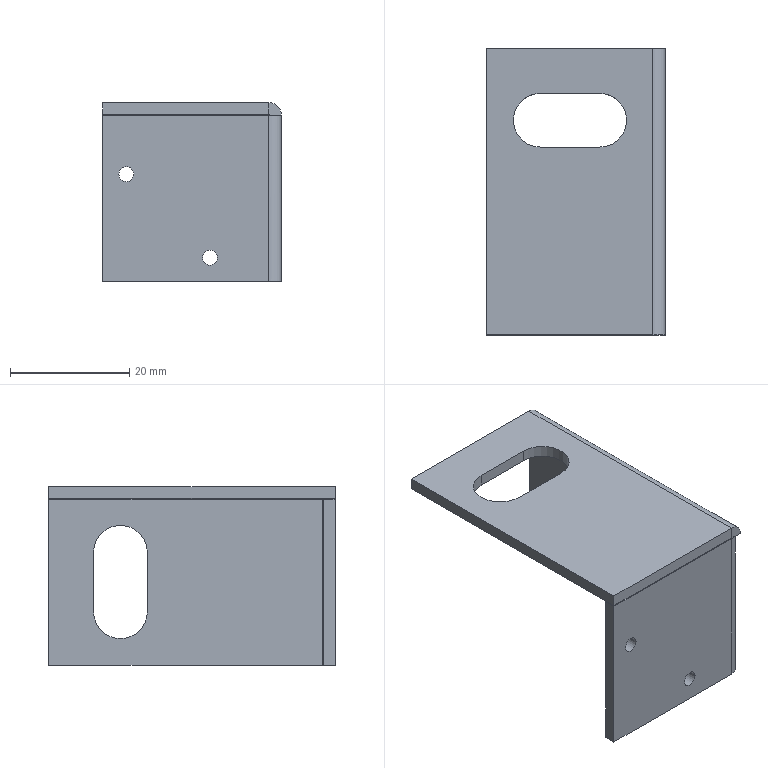Component | SolidWorks | LowerSealingPlateWeldingDrawingPG50-07-1_PG50-07-102(LowerCoverPlateWeldment2)-1 | 1 solid | 36 faces | box 30 x 48 x 30 mm | volume 6419 mm3 | plane 23 | cylinder 13 | commonest cylinder face diameters 9 x5 2.5 x4 0.3 x2 4.3 x2 | material AISI 1045 Steel, cold drawn
STEP:
#1=COLOUR_RGB('',0.7922,0.8196,0.9333);
#2=FILL_AREA_STYLE_COLOUR('',#1);
#3=FILL_AREA_STYLE('',(#2));
#4=SURFACE_STYLE_FILL_AREA(#3);
#5=SURFACE_SIDE_STYLE('',(#4));
#6=SURFACE_STYLE_USAGE(.BOTH.,#5);
#7=PRESENTATION_STYLE_ASSIGNMENT((#6));
#8=CARTESIAN_POINT('',(37.64,-11.134,13.484));
#9=VERTEX_POINT('',#8);
#10=CARTESIAN_POINT('',(37.542,-11.134,13.484));
#11=VERTEX_POINT('',#10);
#12=CARTESIAN_POINT('',(37.591,-11.134,13.484));
#13=DIRECTION('',(-0.,1.,0.));
#14=DIRECTION('',(-1.,0.,0.));
#15=AXIS2_PLACEMENT_3D('',#12,#13,#14);
#16=CIRCLE('',#15,0.04921);
#17=EDGE_CURVE('',#9,#11,#16,.T.);
#18=ORIENTED_EDGE('',*,*,#17,.F.);
#19=CARTESIAN_POINT('',(37.64,-11.055,13.484));
#20=VERTEX_POINT('',#19);
#21=CARTESIAN_POINT('',(37.64,-11.449,13.484));
#22=DIRECTION('',(0.,1.,0.));
#23=VECTOR('',#22,39.37);
#24=LINE('',#21,#23);
#25=EDGE_CURVE('',#9,#20,#24,.T.);
#26=ORIENTED_EDGE('',*,*,#25,.T.);
#27=CARTESIAN_POINT('',(37.542,-11.055,13.484));
#28=VERTEX_POINT('',#27);
#29=CARTESIAN_POINT('',(37.591,-11.055,13.484));
#30=DIRECTION('',(0.,1.,0.));
#31=DIRECTION('',(-1.,0.,0.));
#32=AXIS2_PLACEMENT_3D('',#29,#30,#31);
#33=CIRCLE('',#32,0.04921);
#34=EDGE_CURVE('',#20,#28,#33,.T.);
#35=ORIENTED_EDGE('',*,*,#34,.T.);
#36=CARTESIAN_POINT('',(37.542,-11.449,13.484));
#37=DIRECTION('',(0.,1.,0.));
#38=VECTOR('',#37,39.37);
#39=LINE('',#36,#38);
#40=EDGE_CURVE('',#11,#28,#39,.T.);
#41=ORIENTED_EDGE('',*,*,#40,.F.);
#42=EDGE_LOOP('',(#18,#26,#35,#41));
#43=FACE_OUTER_BOUND('',#42,.T.);
#44=CARTESIAN_POINT('',(37.591,-11.449,13.484));
#45=DIRECTION('',(0.,1.,0.));
#46=DIRECTION('',(-1.,0.,0.));
#47=AXIS2_PLACEMENT_3D('',#44,#45,#46);
#48=CYLINDRICAL_SURFACE('',#47,0.04921);
#49=ADVANCED_FACE('',(#43),#48,.F.);
#50=CARTESIAN_POINT('',(38.192,-11.134,12.933));
#51=VERTEX_POINT('',#50);
#52=CARTESIAN_POINT('',(38.093,-11.134,12.933));
#53=VERTEX_POINT('',#52);
#54=CARTESIAN_POINT('',(38.142,-11.134,12.933));
#55=DIRECTION('',(-0.,1.,0.));
#56=DIRECTION('',(-1.,0.,0.));
#57=AXIS2_PLACEMENT_3D('',#54,#55,#56);
#58=CIRCLE('',#57,0.04921);
#59=EDGE_CURVE('',#51,#53,#58,.T.);
#60=ORIENTED_EDGE('',*,*,#59,.F.);
#61=CARTESIAN_POINT('',(38.192,-11.055,12.933));
#62=VERTEX_POINT('',#61);
#63=CARTESIAN_POINT('',(38.192,-11.449,12.933));
#64=DIRECTION('',(0.,1.,0.));
#65=VECTOR('',#64,39.37);
#66=LINE('',#63,#65);
#67=EDGE_CURVE('',#51,#62,#66,.T.);
#68=ORIENTED_EDGE('',*,*,#67,.T.);
#69=CARTESIAN_POINT('',(38.093,-11.055,12.933));
#70=VERTEX_POINT('',#69);
#71=CARTESIAN_POINT('',(38.142,-11.055,12.933));
#72=DIRECTION('',(0.,1.,0.));
#73=DIRECTION('',(-1.,0.,0.));
#74=AXIS2_PLACEMENT_3D('',#71,#72,#73);
#75=CIRCLE('',#74,0.04921);
#76=EDGE_CURVE('',#62,#70,#75,.T.);
#77=ORIENTED_EDGE('',*,*,#76,.T.);
#78=CARTESIAN_POINT('',(38.093,-11.449,12.933));
#79=DIRECTION('',(0.,1.,0.));
#80=VECTOR('',#79,39.37);
#81=LINE('',#78,#80);
#82=EDGE_CURVE('',#53,#70,#81,.T.);
#83=ORIENTED_EDGE('',*,*,#82,.F.);
#84=EDGE_LOOP('',(#60,#68,#77,#83));
#85=FACE_OUTER_BOUND('',#84,.T.);
#86=CARTESIAN_POINT('',(38.142,-11.449,12.933));
#87=DIRECTION('',(0.,1.,0.));
#88=DIRECTION('',(-1.,0.,0.));
#89=AXIS2_PLACEMENT_3D('',#86,#87,#88);
#90=CYLINDRICAL_SURFACE('',#89,0.04921);
#91=ADVANCED_FACE('',(#85),#90,.F.);
#92=CARTESIAN_POINT('',(38.536,-9.539,13.13));
#93=VERTEX_POINT('',#92);
#94=CARTESIAN_POINT('',(38.536,-9.716,12.953));
#95=VERTEX_POINT('',#94);
#96=CARTESIAN_POINT('',(38.536,-9.716,13.13));
#97=DIRECTION('',(-1.,0.,0.));
#98=DIRECTION('',(0.,-0.,1.));
#99=AXIS2_PLACEMENT_3D('',#96,#97,#98);
#100=CIRCLE('',#99,0.1772);
#101=EDGE_CURVE('',#93,#95,#100,.T.);
#102=ORIENTED_EDGE('',*,*,#101,.T.);
#103=CARTESIAN_POINT('',(38.615,-9.716,12.953));
#104=VERTEX_POINT('',#103);
#105=CARTESIAN_POINT('',(38.221,-9.716,12.953));
#106=DIRECTION('',(1.,-0.,-0.));
#107=VECTOR('',#106,39.37);
#108=LINE('',#105,#107);
#109=EDGE_CURVE('',#95,#104,#108,.T.);
#110=ORIENTED_EDGE('',*,*,#109,.T.);
#111=CARTESIAN_POINT('',(38.615,-9.539,13.13));
#112=VERTEX_POINT('',#111);
#113=CARTESIAN_POINT('',(38.615,-9.716,13.13));
#114=DIRECTION('',(1.,-0.,-0.));
#115=DIRECTION('',(0.,0.,-1.));
#116=AXIS2_PLACEMENT_3D('',#113,#114,#115);
#117=CIRCLE('',#116,0.1772);
#118=EDGE_CURVE('',#104,#112,#117,.T.);
#119=ORIENTED_EDGE('',*,*,#118,.T.);
#120=CARTESIAN_POINT('',(38.221,-9.539,13.13));
#121=DIRECTION('',(1.,-0.,-0.));
#122=VECTOR('',#121,39.37);
#123=LINE('',#120,#122);
#124=EDGE_CURVE('',#93,#112,#123,.T.);
#125=ORIENTED_EDGE('',*,*,#124,.F.);
#126=EDGE_LOOP('',(#102,#110,#119,#125));
#127=FACE_OUTER_BOUND('',#126,.T.);
#128=CARTESIAN_POINT('',(38.221,-9.716,13.13));
#129=DIRECTION('',(1.,-0.,-0.));
#130=DIRECTION('',(0.,0.,-1.));
#131=AXIS2_PLACEMENT_3D('',#128,#129,#130);
#132=CYLINDRICAL_SURFACE('',#131,0.1772);
#133=ADVANCED_FACE('',(#127),#132,.F.);
#134=CARTESIAN_POINT('',(38.536,-11.134,13.872));
#135=VERTEX_POINT('',#134);
#136=CARTESIAN_POINT('',(38.536,-11.134,13.872));
#137=VERTEX_POINT('',#136);
#138=CARTESIAN_POINT('',(38.536,-11.134,13.872));
#139=DIRECTION('',(-0.,1.,0.));
#140=VECTOR('',#139,39.37);
#141=LINE('',#138,#140);
#142=EDGE_CURVE('',#135,#137,#141,.T.);
#143=ORIENTED_EDGE('',*,*,#142,.T.);
#144=CARTESIAN_POINT('',(38.615,-11.049,13.872));
#145=VERTEX_POINT('',#144);
#146=CARTESIAN_POINT('',(38.53,-11.049,13.872));
#147=DIRECTION('',(0.,-0.,1.));
#148=DIRECTION('',(0.,1.,0.));
#149=AXIS2_PLACEMENT_3D('',#146,#147,#148);
#150=CIRCLE('',#149,0.08465);
#151=EDGE_CURVE('',#137,#145,#150,.T.);
#152=ORIENTED_EDGE('',*,*,#151,.T.);
#153=CARTESIAN_POINT('',(38.615,-11.134,13.872));
#154=VERTEX_POINT('',#153);
#155=CARTESIAN_POINT('',(38.615,-9.244,13.872));
#156=DIRECTION('',(-0.,-1.,-0.));
#157=VECTOR('',#156,39.37);
#158=LINE('',#155,#157);
#159=EDGE_CURVE('',#145,#154,#158,.T.);
#160=ORIENTED_EDGE('',*,*,#159,.T.);
#161=CARTESIAN_POINT('',(38.615,-11.134,13.872));
#162=DIRECTION('',(-1.,0.,0.));
#163=VECTOR('',#162,39.37);
#164=LINE('',#161,#163);
#165=EDGE_CURVE('',#154,#135,#164,.T.);
#166=ORIENTED_EDGE('',*,*,#165,.T.);
#167=EDGE_LOOP('',(#143,#152,#160,#166));
#168=FACE_OUTER_BOUND('',#167,.T.);
#169=CARTESIAN_POINT('',(38.536,-11.134,13.872));
#170=DIRECTION('',(-0.,0.,-1.));
#171=DIRECTION('',(-0.,-1.,-0.));
#172=AXIS2_PLACEMENT_3D('',#169,#170,#171);
#173=PLANE('',#172);
#174=ADVANCED_FACE('',(#168),#173,.T.);
#175=CARTESIAN_POINT('',(38.615,-9.894,13.524));
#176=VERTEX_POINT('',#175);
#177=CARTESIAN_POINT('',(38.615,-9.894,13.13));
#178=VERTEX_POINT('',#177);
#179=CARTESIAN_POINT('',(38.615,-9.894,13.13));
#180=DIRECTION('',(-0.,0.,-1.));
#181=VECTOR('',#180,39.37);
#182=LINE('',#179,#181);
#183=EDGE_CURVE('',#176,#178,#182,.T.);
#184=ORIENTED_EDGE('',*,*,#183,.F.);
#185=CARTESIAN_POINT('',(38.615,-9.539,13.524));
#186=VERTEX_POINT('',#185);
#187=CARTESIAN_POINT('',(38.615,-9.716,13.524));
#188=DIRECTION('',(1.,-0.,-0.));
#189=DIRECTION('',(0.,0.,-1.));
#190=AXIS2_PLACEMENT_3D('',#187,#188,#189);
#191=CIRCLE('',#190,0.1772);
#192=EDGE_CURVE('',#186,#176,#191,.T.);
#193=ORIENTED_EDGE('',*,*,#192,.F.);
#194=CARTESIAN_POINT('',(38.615,-9.539,13.524));
#195=DIRECTION('',(0.,-0.,1.));
#196=VECTOR('',#195,39.37);
#197=LINE('',#194,#196);
#198=EDGE_CURVE('',#112,#186,#197,.T.);
#199=ORIENTED_EDGE('',*,*,#198,.F.);
#200=ORIENTED_EDGE('',*,*,#118,.F.);
#201=CARTESIAN_POINT('',(38.615,-9.716,13.13));
#202=DIRECTION('',(1.,-0.,-0.));
#203=DIRECTION('',(0.,0.,-1.));
#204=AXIS2_PLACEMENT_3D('',#201,#202,#203);
#205=CIRCLE('',#204,0.1772);
#206=EDGE_CURVE('',#178,#104,#205,.T.);
#207=ORIENTED_EDGE('',*,*,#206,.F.);
#208=EDGE_LOOP('',(#184,#193,#199,#200,#207));
#209=FACE_BOUND('',#208,.T.);
#210=CARTESIAN_POINT('',(38.615,-11.049,12.776));
#211=VERTEX_POINT('',#210);
#212=CARTESIAN_POINT('',(38.615,-11.049,13.872));
#213=DIRECTION('',(-0.,0.,-1.));
#214=VECTOR('',#213,39.37);
#215=LINE('',#212,#214);
#216=EDGE_CURVE('',#145,#211,#215,.T.);
#217=ORIENTED_EDGE('',*,*,#216,.T.);
#218=CARTESIAN_POINT('',(38.615,-9.244,12.776));
#219=VERTEX_POINT('',#218);
#220=CARTESIAN_POINT('',(38.615,-9.244,12.776));
#221=DIRECTION('',(-0.,-1.,-0.));
#222=VECTOR('',#221,39.37);
#223=LINE('',#220,#222);
#224=EDGE_CURVE('',#219,#211,#223,.T.);
#225=ORIENTED_EDGE('',*,*,#224,.F.);
#226=CARTESIAN_POINT('',(38.615,-9.244,13.872));
#227=VERTEX_POINT('',#226);
#228=CARTESIAN_POINT('',(38.615,-9.244,13.957));
#229=DIRECTION('',(-0.,0.,-1.));
#230=VECTOR('',#229,39.37);
#231=LINE('',#228,#230);
#232=EDGE_CURVE('',#227,#219,#231,.T.);
#233=ORIENTED_EDGE('',*,*,#232,.F.);
#234=CARTESIAN_POINT('',(38.615,-9.244,13.872));
#235=DIRECTION('',(-0.,-1.,-0.));
#236=VECTOR('',#235,39.37);
#237=LINE('',#234,#236);
#238=EDGE_CURVE('',#227,#145,#237,.T.);
#239=ORIENTED_EDGE('',*,*,#238,.T.);
#240=EDGE_LOOP('',(#217,#225,#233,#239));
#241=FACE_OUTER_BOUND('',#240,.T.);
#242=CARTESIAN_POINT('',(38.615,-9.244,13.957));
#243=DIRECTION('',(-1.,0.,0.));
#244=DIRECTION('',(0.,-0.,1.));
#245=AXIS2_PLACEMENT_3D('',#242,#243,#244);
#246=PLANE('',#245);
#247=ADVANCED_FACE('',(#209,#241),#246,.F.);
#248=CARTESIAN_POINT('',(38.536,-9.894,13.524));
#249=VERTEX_POINT('',#248);
#250=CARTESIAN_POINT('',(38.536,-9.539,13.524));
#251=VERTEX_POINT('',#250);
#252=CARTESIAN_POINT('',(38.536,-9.716,13.524));
#253=DIRECTION('',(-1.,0.,0.));
#254=DIRECTION('',(0.,-0.,1.));
#255=AXIS2_PLACEMENT_3D('',#252,#253,#254);
#256=CIRCLE('',#255,0.1772);
#257=EDGE_CURVE('',#249,#251,#256,.T.);
#258=ORIENTED_EDGE('',*,*,#257,.F.);
#259=CARTESIAN_POINT('',(38.536,-9.894,13.13));
#260=VERTEX_POINT('',#259);
#261=CARTESIAN_POINT('',(38.536,-9.894,13.957));
#262=DIRECTION('',(0.,-0.,1.));
#263=VECTOR('',#262,39.37);
#264=LINE('',#261,#263);
#265=EDGE_CURVE('',#260,#249,#264,.T.);
#266=ORIENTED_EDGE('',*,*,#265,.F.);
#267=CARTESIAN_POINT('',(38.536,-9.716,13.13));
#268=DIRECTION('',(-1.,0.,0.));
#269=DIRECTION('',(0.,-0.,1.));
#270=AXIS2_PLACEMENT_3D('',#267,#268,#269);
#271=CIRCLE('',#270,0.1772);
#272=EDGE_CURVE('',#95,#260,#271,.T.);
#273=ORIENTED_EDGE('',*,*,#272,.F.);
#274=ORIENTED_EDGE('',*,*,#101,.F.);
#275=CARTESIAN_POINT('',(38.536,-9.539,13.957));
#276=DIRECTION('',(-0.,0.,-1.));
#277=VECTOR('',#276,39.37);
#278=LINE('',#275,#277);
#279=EDGE_CURVE('',#251,#93,#278,.T.);
#280=ORIENTED_EDGE('',*,*,#279,.F.);
#281=EDGE_LOOP('',(#258,#266,#273,#274,#280));
#282=FACE_BOUND('',#281,.T.);
#283=CARTESIAN_POINT('',(38.536,-9.244,12.776));
#284=VERTEX_POINT('',#283);
#285=CARTESIAN_POINT('',(38.536,-11.049,12.776));
#286=VERTEX_POINT('',#285);
#287=CARTESIAN_POINT('',(38.536,-9.244,12.776));
#288=DIRECTION('',(-0.,-1.,-0.));
#289=VECTOR('',#288,39.37);
#290=LINE('',#287,#289);
#291=EDGE_CURVE('',#284,#286,#290,.T.);
#292=ORIENTED_EDGE('',*,*,#291,.T.);
#293=CARTESIAN_POINT('',(38.536,-11.049,13.872));
#294=VERTEX_POINT('',#293);
#295=CARTESIAN_POINT('',(38.536,-11.049,13.872));
#296=DIRECTION('',(-0.,0.,-1.));
#297=VECTOR('',#296,39.37);
#298=LINE('',#295,#297);
#299=EDGE_CURVE('',#294,#286,#298,.T.);
#300=ORIENTED_EDGE('',*,*,#299,.F.);
#301=CARTESIAN_POINT('',(38.536,-9.244,13.872));
#302=VERTEX_POINT('',#301);
#303=CARTESIAN_POINT('',(38.536,-9.244,13.872));
#304=DIRECTION('',(-0.,-1.,-0.));
#305=VECTOR('',#304,39.37);
#306=LINE('',#303,#305);
#307=EDGE_CURVE('',#302,#294,#306,.T.);
#308=ORIENTED_EDGE('',*,*,#307,.F.);
#309=CARTESIAN_POINT('',(38.536,-9.244,13.957));
#310=DIRECTION('',(-0.,0.,-1.));
#311=VECTOR('',#310,39.37);
#312=LINE('',#309,#311);
#313=EDGE_CURVE('',#302,#284,#312,.T.);
#314=ORIENTED_EDGE('',*,*,#313,.T.);
#315=EDGE_LOOP('',(#292,#300,#308,#314));
#316=FACE_OUTER_BOUND('',#315,.T.);
#317=CARTESIAN_POINT('',(38.536,-9.244,13.957));
#318=DIRECTION('',(-1.,0.,0.));
#319=DIRECTION('',(0.,-0.,1.));
#320=AXIS2_PLACEMENT_3D('',#317,#318,#319);
#321=PLANE('',#320);
#322=ADVANCED_FACE('',(#282,#316),#321,.T.);
#323=CARTESIAN_POINT('',(38.53,-9.244,13.957));
#324=VERTEX_POINT('',#323);
#325=CARTESIAN_POINT('',(38.53,-9.244,13.878));
#326=VERTEX_POINT('',#325);
#327=CARTESIAN_POINT('',(38.53,-9.244,13.957));
#328=DIRECTION('',(-0.,0.,-1.));
#329=VECTOR('',#328,39.37);
#330=LINE('',#327,#329);
#331=EDGE_CURVE('',#324,#326,#330,.T.);
#332=ORIENTED_EDGE('',*,*,#331,.F.);
#333=CARTESIAN_POINT('',(38.53,-9.244,13.872));
#334=DIRECTION('',(0.,1.,0.));
#335=DIRECTION('',(1.,0.,0.));
#336=AXIS2_PLACEMENT_3D('',#333,#334,#335);
#337=CIRCLE('',#336,0.08465);
#338=EDGE_CURVE('',#324,#227,#337,.T.);
#339=ORIENTED_EDGE('',*,*,#338,.T.);
#340=CARTESIAN_POINT('',(38.536,-9.244,13.872));
#341=DIRECTION('',(1.,-0.,-0.));
#342=VECTOR('',#341,39.37);
#343=LINE('',#340,#342);
#344=EDGE_CURVE('',#302,#227,#343,.T.);
#345=ORIENTED_EDGE('',*,*,#344,.F.);
#346=CARTESIAN_POINT('',(38.53,-9.244,13.872));
#347=DIRECTION('',(0.,1.,0.));
#348=DIRECTION('',(-1.,0.,0.));
#349=AXIS2_PLACEMENT_3D('',#346,#347,#348);
#350=CIRCLE('',#349,0.005906);
#351=EDGE_CURVE('',#326,#302,#350,.T.);
#352=ORIENTED_EDGE('',*,*,#351,.F.);
#353=EDGE_LOOP('',(#332,#339,#345,#352));
#354=FACE_OUTER_BOUND('',#353,.T.);
#355=CARTESIAN_POINT('',(38.53,-9.244,13.957));
#356=DIRECTION('',(0.,1.,0.));
#357=DIRECTION('',(-1.,0.,0.));
#358=AXIS2_PLACEMENT_3D('',#355,#356,#357);
#359=PLANE('',#358);
#360=ADVANCED_FACE('',(#354),#359,.T.);
#361=CARTESIAN_POINT('',(37.434,-9.244,13.957));
#362=VERTEX_POINT('',#361);
#363=CARTESIAN_POINT('',(38.615,-9.244,13.957));
#364=DIRECTION('',(1.,-0.,-0.));
#365=VECTOR('',#364,39.37);
#366=LINE('',#363,#365);
#367=EDGE_CURVE('',#362,#324,#366,.T.);
#368=ORIENTED_EDGE('',*,*,#367,.T.);
#369=ORIENTED_EDGE('',*,*,#331,.T.);
#370=CARTESIAN_POINT('',(37.434,-9.244,13.878));
#371=VERTEX_POINT('',#370);
#372=CARTESIAN_POINT('',(38.615,-9.244,13.878));
#373=DIRECTION('',(1.,-0.,-0.));
#374=VECTOR('',#373,39.37);
#375=LINE('',#372,#374);
#376=EDGE_CURVE('',#371,#326,#375,.T.);
#377=ORIENTED_EDGE('',*,*,#376,.F.);
#378=CARTESIAN_POINT('',(37.434,-9.244,13.957));
#379=DIRECTION('',(-0.,0.,-1.));
#380=VECTOR('',#379,39.37);
#381=LINE('',#378,#380);
#382=EDGE_CURVE('',#362,#371,#381,.T.);
#383=ORIENTED_EDGE('',*,*,#382,.F.);
#384=EDGE_LOOP('',(#368,#369,#377,#383));
#385=FACE_OUTER_BOUND('',#384,.T.);
#386=CARTESIAN_POINT('',(38.536,-9.244,13.872));
#387=DIRECTION('',(0.,1.,0.));
#388=DIRECTION('',(-1.,0.,0.));
#389=AXIS2_PLACEMENT_3D('',#386,#387,#388);
#390=PLANE('',#389);
#391=ADVANCED_FACE('',(#385),#390,.T.);
#392=ORIENTED_EDGE('',*,*,#165,.F.);
#393=CARTESIAN_POINT('',(38.53,-11.134,13.957));
#394=VERTEX_POINT('',#393);
#395=CARTESIAN_POINT('',(38.53,-11.134,13.872));
#396=DIRECTION('',(0.,1.,0.));
#397=DIRECTION('',(1.,0.,0.));
#398=AXIS2_PLACEMENT_3D('',#395,#396,#397);
#399=CIRCLE('',#398,0.08465);
#400=EDGE_CURVE('',#394,#154,#399,.T.);
#401=ORIENTED_EDGE('',*,*,#400,.F.);
#402=CARTESIAN_POINT('',(38.53,-11.134,13.878));
#403=VERTEX_POINT('',#402);
#404=CARTESIAN_POINT('',(38.53,-11.134,13.878));
#405=DIRECTION('',(0.,-0.,1.));
#406=VECTOR('',#405,39.37);
#407=LINE('',#404,#406);
#408=EDGE_CURVE('',#403,#394,#407,.T.);
#409=ORIENTED_EDGE('',*,*,#408,.F.);
#410=CARTESIAN_POINT('',(38.53,-11.134,13.872));
#411=DIRECTION('',(0.,1.,0.));
#412=DIRECTION('',(-1.,0.,0.));
#413=AXIS2_PLACEMENT_3D('',#410,#411,#412);
#414=CIRCLE('',#413,0.005906);
#415=EDGE_CURVE('',#403,#135,#414,.T.);
#416=ORIENTED_EDGE('',*,*,#415,.T.);
#417=EDGE_LOOP('',(#392,#401,#409,#416));
#418=FACE_OUTER_BOUND('',#417,.T.);
#419=CARTESIAN_POINT('',(38.615,-11.134,13.872));
#420=DIRECTION('',(-0.,-1.,-0.));
#421=DIRECTION('',(1.,-0.,-0.));
#422=AXIS2_PLACEMENT_3D('',#419,#420,#421);
#423=PLANE('',#422);
#424=ADVANCED_FACE('',(#418),#423,.T.);
#425=CARTESIAN_POINT('',(38.536,-11.049,12.776));
#426=DIRECTION('',(1.,-0.,-0.));
#427=VECTOR('',#426,39.37);
#428=LINE('',#425,#427);
#429=EDGE_CURVE('',#286,#211,#428,.T.);
#430=ORIENTED_EDGE('',*,*,#429,.F.);
#431=ORIENTED_EDGE('',*,*,#291,.F.);
#432=CARTESIAN_POINT('',(38.536,-9.244,12.776));
#433=DIRECTION('',(1.,-0.,-0.));
#434=VECTOR('',#433,39.37);
#435=LINE('',#432,#434);
#436=EDGE_CURVE('',#284,#219,#435,.T.);
#437=ORIENTED_EDGE('',*,*,#436,.T.);
#438=ORIENTED_EDGE('',*,*,#224,.T.);
#439=EDGE_LOOP('',(#430,#431,#437,#438));
#440=FACE_OUTER_BOUND('',#439,.T.);
#441=CARTESIAN_POINT('',(38.536,-9.244,12.776));
#442=DIRECTION('',(-0.,0.,-1.));
#443=DIRECTION('',(-0.,-1.,-0.));
#444=AXIS2_PLACEMENT_3D('',#441,#442,#443);
#445=PLANE('',#444);
#446=ADVANCED_FACE('',(#440),#445,.T.);
#447=ORIENTED_EDGE('',*,*,#415,.F.);
#448=CARTESIAN_POINT('',(38.53,-9.244,13.878));
#449=DIRECTION('',(-0.,-1.,-0.));
#450=VECTOR('',#449,39.37);
#451=LINE('',#448,#450);
#452=EDGE_CURVE('',#326,#403,#451,.T.);
#453=ORIENTED_EDGE('',*,*,#452,.F.);
#454=ORIENTED_EDGE('',*,*,#351,.T.);
#455=ORIENTED_EDGE('',*,*,#307,.T.);
#456=CARTESIAN_POINT('',(38.536,-11.134,13.872));
#457=DIRECTION('',(-0.,1.,0.));
#458=VECTOR('',#457,39.37);
#459=LINE('',#456,#458);
#460=EDGE_CURVE('',#137,#294,#459,.T.);
#461=ORIENTED_EDGE('',*,*,#460,.F.);
#462=ORIENTED_EDGE('',*,*,#142,.F.);
#463=EDGE_LOOP('',(#447,#453,#454,#455,#461,#462));
#464=FACE_OUTER_BOUND('',#463,.T.);
#465=CARTESIAN_POINT('',(38.53,-9.244,13.872));
#466=DIRECTION('',(-0.,-1.,-0.));
#467=DIRECTION('',(1.,0.,0.));
#468=AXIS2_PLACEMENT_3D('',#465,#466,#467);
#469=CYLINDRICAL_SURFACE('',#468,0.005906);
#470=ADVANCED_FACE('',(#464),#469,.F.);
#471=CARTESIAN_POINT('',(37.788,-9.894,13.878));
#472=VERTEX_POINT('',#471);
#473=CARTESIAN_POINT('',(37.788,-9.539,13.878));
#474=VERTEX_POINT('',#473);
#475=CARTESIAN_POINT('',(37.788,-9.716,13.878));
#476=DIRECTION('',(-0.,0.,-1.));
#477=DIRECTION('',(0.,-1.,0.));
#478=AXIS2_PLACEMENT_3D('',#475,#476,#477);
#479=CIRCLE('',#478,0.1772);
#480=EDGE_CURVE('',#472,#474,#479,.T.);
#481=ORIENTED_EDGE('',*,*,#480,.F.);
#482=CARTESIAN_POINT('',(38.182,-9.894,13.878));
#483=VERTEX_POINT('',#482);
#484=CARTESIAN_POINT('',(38.182,-9.894,13.878));
#485=DIRECTION('',(-1.,0.,0.));
#486=VECTOR('',#485,39.37);
#487=LINE('',#484,#486);
#488=EDGE_CURVE('',#483,#472,#487,.T.);
#489=ORIENTED_EDGE('',*,*,#488,.F.);
#490=CARTESIAN_POINT('',(38.182,-9.539,13.878));
#491=VERTEX_POINT('',#490);
#492=CARTESIAN_POINT('',(38.182,-9.716,13.878));
#493=DIRECTION('',(-0.,0.,-1.));
#494=DIRECTION('',(0.,-1.,0.));
#495=AXIS2_PLACEMENT_3D('',#492,#493,#494);
#496=CIRCLE('',#495,0.1772);
#497=EDGE_CURVE('',#491,#483,#496,.T.);
#498=ORIENTED_EDGE('',*,*,#497,.F.);
#499=CARTESIAN_POINT('',(37.788,-9.539,13.878));
#500=DIRECTION('',(1.,-0.,-0.));
#501=VECTOR('',#500,39.37);
#502=LINE('',#499,#501);
#503=EDGE_CURVE('',#474,#491,#502,.T.);
#504=ORIENTED_EDGE('',*,*,#503,.F.);
#505=EDGE_LOOP('',(#481,#489,#498,#504));
#506=FACE_BOUND('',#505,.T.);
#507=CARTESIAN_POINT('',(37.434,-11.134,13.878));
#508=VERTEX_POINT('',#507);
#509=CARTESIAN_POINT('',(38.615,-11.134,13.878));
#510=DIRECTION('',(1.,-0.,-0.));
#511=VECTOR('',#510,39.37);
#512=LINE('',#509,#511);
#513=EDGE_CURVE('',#508,#403,#512,.T.);
#514=ORIENTED_EDGE('',*,*,#513,.F.);
#515=CARTESIAN_POINT('',(37.434,-9.244,13.878));
#516=DIRECTION('',(-0.,-1.,-0.));
#517=VECTOR('',#516,39.37);
#518=LINE('',#515,#517);
#519=EDGE_CURVE('',#371,#508,#518,.T.);
#520=ORIENTED_EDGE('',*,*,#519,.F.);
#521=ORIENTED_EDGE('',*,*,#376,.T.);
#522=ORIENTED_EDGE('',*,*,#452,.T.);
#523=EDGE_LOOP('',(#514,#520,#521,#522));
#524=FACE_OUTER_BOUND('',#523,.T.);
#525=CARTESIAN_POINT('',(38.615,-9.244,13.878));
#526=DIRECTION('',(-0.,0.,-1.));
#527=DIRECTION('',(-0.,-1.,-0.));
#528=AXIS2_PLACEMENT_3D('',#525,#526,#527);
#529=PLANE('',#528);
#530=ADVANCED_FACE('',(#506,#524),#529,.T.);
#531=CARTESIAN_POINT('',(37.434,-11.134,13.957));
#532=VERTEX_POINT('',#531);
#533=CARTESIAN_POINT('',(37.434,-11.134,13.957));
#534=DIRECTION('',(-0.,0.,-1.));
#535=VECTOR('',#534,39.37);
#536=LINE('',#533,#535);
#537=EDGE_CURVE('',#532,#508,#536,.T.);
#538=ORIENTED_EDGE('',*,*,#537,.F.);
#539=CARTESIAN_POINT('',(37.434,-9.244,13.957));
#540=DIRECTION('',(-0.,-1.,-0.));
#541=VECTOR('',#540,39.37);
#542=LINE('',#539,#541);
#543=EDGE_CURVE('',#362,#532,#542,.T.);
#544=ORIENTED_EDGE('',*,*,#543,.F.);
#545=ORIENTED_EDGE('',*,*,#382,.T.);
#546=ORIENTED_EDGE('',*,*,#519,.T.);
#547=EDGE_LOOP('',(#538,#544,#545,#546));
#548=FACE_OUTER_BOUND('',#547,.T.);
#549=CARTESIAN_POINT('',(37.434,-9.244,13.957));
#550=DIRECTION('',(-1.,0.,0.));
#551=DIRECTION('',(-0.,-1.,-0.));
#552=AXIS2_PLACEMENT_3D('',#549,#550,#551);
#553=PLANE('',#552);
#554=ADVANCED_FACE('',(#548),#553,.T.);
#555=CARTESIAN_POINT('',(38.182,-9.894,13.957));
#556=VERTEX_POINT('',#555);
#557=CARTESIAN_POINT('',(37.788,-9.894,13.957));
#558=VERTEX_POINT('',#557);
#559=CARTESIAN_POINT('',(38.615,-9.894,13.957));
#560=DIRECTION('',(-1.,0.,0.));
#561=VECTOR('',#560,39.37);
#562=LINE('',#559,#561);
#563=EDGE_CURVE('',#556,#558,#562,.T.);
#564=ORIENTED_EDGE('',*,*,#563,.T.);
#565=CARTESIAN_POINT('',(37.788,-9.539,13.957));
#566=VERTEX_POINT('',#565);
#567=CARTESIAN_POINT('',(37.788,-9.716,13.957));
#568=DIRECTION('',(-0.,0.,-1.));
#569=DIRECTION('',(0.,-1.,0.));
#570=AXIS2_PLACEMENT_3D('',#567,#568,#569);
#571=CIRCLE('',#570,0.1772);
#572=EDGE_CURVE('',#558,#566,#571,.T.);
#573=ORIENTED_EDGE('',*,*,#572,.T.);
#574=CARTESIAN_POINT('',(38.182,-9.539,13.957));
#575=VERTEX_POINT('',#574);
#576=CARTESIAN_POINT('',(38.615,-9.539,13.957));
#577=DIRECTION('',(1.,-0.,-0.));
#578=VECTOR('',#577,39.37);
#579=LINE('',#576,#578);
#580=EDGE_CURVE('',#566,#575,#579,.T.);
#581=ORIENTED_EDGE('',*,*,#580,.T.);
#582=CARTESIAN_POINT('',(38.182,-9.716,13.957));
#583=DIRECTION('',(-0.,0.,-1.));
#584=DIRECTION('',(0.,-1.,0.));
#585=AXIS2_PLACEMENT_3D('',#582,#583,#584);
#586=CIRCLE('',#585,0.1772);
#587=EDGE_CURVE('',#575,#556,#586,.T.);
#588=ORIENTED_EDGE('',*,*,#587,.T.);
#589=EDGE_LOOP('',(#564,#573,#581,#588));
#590=FACE_BOUND('',#589,.T.);
#591=CARTESIAN_POINT('',(38.615,-11.134,13.957));
#592=DIRECTION('',(1.,-0.,-0.));
#593=VECTOR('',#592,39.37);
#594=LINE('',#591,#593);
#595=EDGE_CURVE('',#532,#394,#594,.T.);
#596=ORIENTED_EDGE('',*,*,#595,.T.);
#597=CARTESIAN_POINT('',(38.53,-9.244,13.957));
#598=DIRECTION('',(-0.,-1.,-0.));
#599=VECTOR('',#598,39.37);
#600=LINE('',#597,#599);
#601=EDGE_CURVE('',#324,#394,#600,.T.);
#602=ORIENTED_EDGE('',*,*,#601,.F.);
#603=ORIENTED_EDGE('',*,*,#367,.F.);
#604=ORIENTED_EDGE('',*,*,#543,.T.);
#605=EDGE_LOOP('',(#596,#602,#603,#604));
#606=FACE_OUTER_BOUND('',#605,.T.);
#607=CARTESIAN_POINT('',(38.615,-9.244,13.957));
#608=DIRECTION('',(-0.,0.,-1.));
#609=DIRECTION('',(-0.,-1.,-0.));
#610=AXIS2_PLACEMENT_3D('',#607,#608,#609);
#611=PLANE('',#610);
#612=ADVANCED_FACE('',(#590,#606),#611,.F.);
#613=ORIENTED_EDGE('',*,*,#400,.T.);
#614=ORIENTED_EDGE('',*,*,#159,.F.);
#615=ORIENTED_EDGE('',*,*,#238,.F.);
#616=ORIENTED_EDGE('',*,*,#338,.F.);
#617=ORIENTED_EDGE('',*,*,#601,.T.);
#618=EDGE_LOOP('',(#613,#614,#615,#616,#617));
#619=FACE_OUTER_BOUND('',#618,.T.);
#620=CARTESIAN_POINT('',(38.53,-9.244,13.872));
#621=DIRECTION('',(-0.,-1.,-0.));
#622=DIRECTION('',(1.,0.,0.));
#623=AXIS2_PLACEMENT_3D('',#620,#621,#622);
#624=CYLINDRICAL_SURFACE('',#623,0.08465);
#625=ADVANCED_FACE('',(#619),#624,.T.);
#626=ORIENTED_EDGE('',*,*,#232,.T.);
#627=ORIENTED_EDGE('',*,*,#436,.F.);
#628=ORIENTED_EDGE('',*,*,#313,.F.);
#629=ORIENTED_EDGE('',*,*,#344,.T.);
#630=EDGE_LOOP('',(#626,#627,#628,#629));
#631=FACE_OUTER_BOUND('',#630,.T.);
#632=CARTESIAN_POINT('',(38.53,-9.244,13.872));
#633=DIRECTION('',(0.,1.,0.));
#634=DIRECTION('',(-1.,0.,0.));
#635=AXIS2_PLACEMENT_3D('',#632,#633,#634);
#636=PLANE('',#635);
#637=ADVANCED_FACE('',(#631),#636,.T.);
#638=ORIENTED_EDGE('',*,*,#513,.T.);
#639=ORIENTED_EDGE('',*,*,#408,.T.);
#640=ORIENTED_EDGE('',*,*,#595,.F.);
#641=ORIENTED_EDGE('',*,*,#537,.T.);
#642=EDGE_LOOP('',(#638,#639,#640,#641));
#643=FACE_OUTER_BOUND('',#642,.T.);
#644=CARTESIAN_POINT('',(38.53,-11.134,13.872));
#645=DIRECTION('',(0.,1.,0.));
#646=DIRECTION('',(-1.,0.,0.));
#647=AXIS2_PLACEMENT_3D('',#644,#645,#646);
#648=PLANE('',#647);
#649=ADVANCED_FACE('',(#643),#648,.F.);
#650=CARTESIAN_POINT('',(38.53,-11.055,12.776));
#651=VERTEX_POINT('',#650);
#652=CARTESIAN_POINT('',(38.53,-11.134,12.776));
#653=VERTEX_POINT('',#652);
#654=CARTESIAN_POINT('',(38.53,-11.134,12.776));
#655=DIRECTION('',(-0.,-1.,-0.));
#656=VECTOR('',#655,39.37);
#657=LINE('',#654,#656);
#658=EDGE_CURVE('',#651,#653,#657,.T.);
#659=ORIENTED_EDGE('',*,*,#658,.F.);
#660=CARTESIAN_POINT('',(38.53,-11.049,12.776));
#661=DIRECTION('',(-0.,0.,-1.));
#662=DIRECTION('',(0.,1.,0.));
#663=AXIS2_PLACEMENT_3D('',#660,#661,#662);
#664=CIRCLE('',#663,0.005906);
#665=EDGE_CURVE('',#286,#651,#664,.T.);
#666=ORIENTED_EDGE('',*,*,#665,.F.);
#667=ORIENTED_EDGE('',*,*,#429,.T.);
#668=CARTESIAN_POINT('',(38.53,-11.049,12.776));
#669=DIRECTION('',(-0.,0.,-1.));
#670=DIRECTION('',(0.,1.,0.));
#671=AXIS2_PLACEMENT_3D('',#668,#669,#670);
#672=CIRCLE('',#671,0.08465);
#673=EDGE_CURVE('',#211,#653,#672,.T.);
#674=ORIENTED_EDGE('',*,*,#673,.T.);
#675=EDGE_LOOP('',(#659,#666,#667,#674));
#676=FACE_OUTER_BOUND('',#675,.T.);
#677=CARTESIAN_POINT('',(38.53,-11.049,12.776));
#678=DIRECTION('',(-0.,0.,-1.));
#679=DIRECTION('',(-0.,-1.,-0.));
#680=AXIS2_PLACEMENT_3D('',#677,#678,#679);
#681=PLANE('',#680);
#682=ADVANCED_FACE('',(#676),#681,.T.);
#683=CARTESIAN_POINT('',(38.53,-11.134,13.872));
#684=VERTEX_POINT('',#683);
#685=CARTESIAN_POINT('',(38.53,-11.049,13.872));
#686=DIRECTION('',(0.,-0.,1.));
#687=DIRECTION('',(0.,1.,0.));
#688=AXIS2_PLACEMENT_3D('',#685,#686,#687);
#689=CIRCLE('',#688,0.08465);
#690=EDGE_CURVE('',#684,#137,#689,.T.);
#691=ORIENTED_EDGE('',*,*,#690,.T.);
#692=ORIENTED_EDGE('',*,*,#460,.T.);
#693=CARTESIAN_POINT('',(38.53,-11.055,13.872));
#694=VERTEX_POINT('',#693);
#695=CARTESIAN_POINT('',(38.53,-11.049,13.872));
#696=DIRECTION('',(0.,-0.,1.));
#697=DIRECTION('',(0.,1.,0.));
#698=AXIS2_PLACEMENT_3D('',#695,#696,#697);
#699=CIRCLE('',#698,0.005906);
#700=EDGE_CURVE('',#694,#294,#699,.T.);
#701=ORIENTED_EDGE('',*,*,#700,.F.);
#702=CARTESIAN_POINT('',(38.53,-11.055,13.872));
#703=DIRECTION('',(-0.,-1.,-0.));
#704=VECTOR('',#703,39.37);
#705=LINE('',#702,#704);
#706=EDGE_CURVE('',#694,#684,#705,.T.);
#707=ORIENTED_EDGE('',*,*,#706,.T.);
#708=EDGE_LOOP('',(#691,#692,#701,#707));
#709=FACE_OUTER_BOUND('',#708,.T.);
#710=CARTESIAN_POINT('',(38.53,-11.049,13.872));
#711=DIRECTION('',(-0.,0.,-1.));
#712=DIRECTION('',(-0.,-1.,-0.));
#713=AXIS2_PLACEMENT_3D('',#710,#711,#712);
#714=PLANE('',#713);
#715=ADVANCED_FACE('',(#709),#714,.F.);
#716=ORIENTED_EDGE('',*,*,#216,.F.);
#717=ORIENTED_EDGE('',*,*,#151,.F.);
#718=ORIENTED_EDGE('',*,*,#690,.F.);
#719=CARTESIAN_POINT('',(38.53,-11.134,12.776));
#720=DIRECTION('',(-0.,0.,-1.));
#721=VECTOR('',#720,39.37);
#722=LINE('',#719,#721);
#723=EDGE_CURVE('',#684,#653,#722,.T.);
#724=ORIENTED_EDGE('',*,*,#723,.T.);
#725=ORIENTED_EDGE('',*,*,#673,.F.);
#726=EDGE_LOOP('',(#716,#717,#718,#724,#725));
#727=FACE_OUTER_BOUND('',#726,.T.);
#728=CARTESIAN_POINT('',(38.53,-11.049,13.872));
#729=DIRECTION('',(0.,-0.,1.));
#730=DIRECTION('',(0.,-1.,0.));
#731=AXIS2_PLACEMENT_3D('',#728,#729,#730);
#732=CYLINDRICAL_SURFACE('',#731,0.08465);
#733=ADVANCED_FACE('',(#727),#732,.T.);
#734=ORIENTED_EDGE('',*,*,#299,.T.);
#735=ORIENTED_EDGE('',*,*,#665,.T.);
#736=CARTESIAN_POINT('',(38.53,-11.055,12.776));
#737=DIRECTION('',(0.,-0.,1.));
#738=VECTOR('',#737,39.37);
#739=LINE('',#736,#738);
#740=EDGE_CURVE('',#651,#694,#739,.T.);
#741=ORIENTED_EDGE('',*,*,#740,.T.);
#742=ORIENTED_EDGE('',*,*,#700,.T.);
#743=EDGE_LOOP('',(#734,#735,#741,#742));
#744=FACE_OUTER_BOUND('',#743,.T.);
#745=CARTESIAN_POINT('',(38.53,-11.049,13.872));
#746=DIRECTION('',(0.,-0.,1.));
#747=DIRECTION('',(0.,-1.,0.));
#748=AXIS2_PLACEMENT_3D('',#745,#746,#747);
#749=CYLINDRICAL_SURFACE('',#748,0.005906);
#750=ADVANCED_FACE('',(#744),#749,.F.);
#751=ORIENTED_EDGE('',*,*,#706,.F.);
#752=CARTESIAN_POINT('',(37.434,-11.055,13.872));
#753=VERTEX_POINT('',#752);
#754=CARTESIAN_POINT('',(37.434,-11.055,13.872));
#755=DIRECTION('',(-1.,-0.,0.));
#756=VECTOR('',#755,39.37);
#757=LINE('',#754,#756);
#758=EDGE_CURVE('',#694,#753,#757,.T.);
#759=ORIENTED_EDGE('',*,*,#758,.T.);
#760=CARTESIAN_POINT('',(37.434,-11.134,13.872));
#761=VERTEX_POINT('',#760);
#762=CARTESIAN_POINT('',(37.434,-11.134,13.872));
#763=DIRECTION('',(-0.,1.,0.));
#764=VECTOR('',#763,39.37);
#765=LINE('',#762,#764);
#766=EDGE_CURVE('',#761,#753,#765,.T.);
#767=ORIENTED_EDGE('',*,*,#766,.F.);
#768=CARTESIAN_POINT('',(38.615,-11.134,13.872));
#769=DIRECTION('',(-1.,-0.,0.));
#770=VECTOR('',#769,39.37);
#771=LINE('',#768,#770);
#772=EDGE_CURVE('',#684,#761,#771,.T.);
#773=ORIENTED_EDGE('',*,*,#772,.F.);
#774=EDGE_LOOP('',(#751,#759,#767,#773));
#775=FACE_OUTER_BOUND('',#774,.T.);
#776=CARTESIAN_POINT('',(37.434,-11.134,13.872));
#777=DIRECTION('',(-0.,0.,-1.));
#778=DIRECTION('',(-1.,0.,0.));
#779=AXIS2_PLACEMENT_3D('',#776,#777,#778);
#780=PLANE('',#779);
#781=ADVANCED_FACE('',(#775),#780,.F.);
#782=ORIENTED_EDGE('',*,*,#658,.T.);
#783=CARTESIAN_POINT('',(37.434,-11.134,12.776));
#784=VERTEX_POINT('',#783);
#785=CARTESIAN_POINT('',(38.615,-11.134,12.776));
#786=DIRECTION('',(1.,0.,-0.));
#787=VECTOR('',#786,39.37);
#788=LINE('',#785,#787);
#789=EDGE_CURVE('',#784,#653,#788,.T.);
#790=ORIENTED_EDGE('',*,*,#789,.F.);
#791=CARTESIAN_POINT('',(37.434,-11.055,12.776));
#792=VERTEX_POINT('',#791);
#793=CARTESIAN_POINT('',(37.434,-11.134,12.776));
#794=DIRECTION('',(-0.,1.,0.));
#795=VECTOR('',#794,39.37);
#796=LINE('',#793,#795);
#797=EDGE_CURVE('',#784,#792,#796,.T.);
#798=ORIENTED_EDGE('',*,*,#797,.T.);
#799=CARTESIAN_POINT('',(38.536,-11.055,12.776));
#800=DIRECTION('',(1.,0.,-0.));
#801=VECTOR('',#800,39.37);
#802=LINE('',#799,#801);
#803=EDGE_CURVE('',#792,#651,#802,.T.);
#804=ORIENTED_EDGE('',*,*,#803,.T.);
#805=EDGE_LOOP('',(#782,#790,#798,#804));
#806=FACE_OUTER_BOUND('',#805,.T.);
#807=CARTESIAN_POINT('',(38.536,-11.134,12.776));
#808=DIRECTION('',(0.,-0.,1.));
#809=DIRECTION('',(1.,-0.,-0.));
#810=AXIS2_PLACEMENT_3D('',#807,#808,#809);
#811=PLANE('',#810);
#812=ADVANCED_FACE('',(#806),#811,.F.);
#813=CARTESIAN_POINT('',(37.591,-11.134,13.484));
#814=DIRECTION('',(-0.,1.,0.));
#815=DIRECTION('',(-1.,0.,0.));
#816=AXIS2_PLACEMENT_3D('',#813,#814,#815);
#817=CIRCLE('',#816,0.04921);
#818=EDGE_CURVE('',#11,#9,#817,.T.);
#819=ORIENTED_EDGE('',*,*,#818,.T.);
#820=ORIENTED_EDGE('',*,*,#17,.T.);
#821=EDGE_LOOP('',(#819,#820));
#822=FACE_BOUND('',#821,.T.);
#823=CARTESIAN_POINT('',(38.142,-11.134,12.933));
#824=DIRECTION('',(-0.,1.,0.));
#825=DIRECTION('',(-1.,0.,0.));
#826=AXIS2_PLACEMENT_3D('',#823,#824,#825);
#827=CIRCLE('',#826,0.04921);
#828=EDGE_CURVE('',#53,#51,#827,.T.);
#829=ORIENTED_EDGE('',*,*,#828,.T.);
#830=ORIENTED_EDGE('',*,*,#59,.T.);
#831=EDGE_LOOP('',(#829,#830));
#832=FACE_BOUND('',#831,.T.);
#833=ORIENTED_EDGE('',*,*,#723,.F.);
#834=ORIENTED_EDGE('',*,*,#772,.T.);
#835=CARTESIAN_POINT('',(37.434,-11.134,13.957));
#836=DIRECTION('',(-0.,0.,-1.));
#837=VECTOR('',#836,39.37);
#838=LINE('',#835,#837);
#839=EDGE_CURVE('',#761,#784,#838,.T.);
#840=ORIENTED_EDGE('',*,*,#839,.T.);
#841=ORIENTED_EDGE('',*,*,#789,.T.);
#842=EDGE_LOOP('',(#833,#834,#840,#841));
#843=FACE_OUTER_BOUND('',#842,.T.);
#844=CARTESIAN_POINT('',(38.615,-11.134,13.957));
#845=DIRECTION('',(-0.,1.,0.));
#846=DIRECTION('',(-1.,-0.,0.));
#847=AXIS2_PLACEMENT_3D('',#844,#845,#846);
#848=PLANE('',#847);
#849=ADVANCED_FACE('',(#822,#832,#843),#848,.F.);
#850=CARTESIAN_POINT('',(37.591,-11.055,13.484));
#851=DIRECTION('',(0.,1.,0.));
#852=DIRECTION('',(-1.,0.,0.));
#853=AXIS2_PLACEMENT_3D('',#850,#851,#852);
#854=CIRCLE('',#853,0.04921);
#855=EDGE_CURVE('',#28,#20,#854,.T.);
#856=ORIENTED_EDGE('',*,*,#855,.F.);
#857=ORIENTED_EDGE('',*,*,#34,.F.);
#858=EDGE_LOOP('',(#856,#857));
#859=FACE_BOUND('',#858,.T.);
#860=CARTESIAN_POINT('',(38.142,-11.055,12.933));
#861=DIRECTION('',(0.,1.,0.));
#862=DIRECTION('',(-1.,0.,0.));
#863=AXIS2_PLACEMENT_3D('',#860,#861,#862);
#864=CIRCLE('',#863,0.04921);
#865=EDGE_CURVE('',#70,#62,#864,.T.);
#866=ORIENTED_EDGE('',*,*,#865,.F.);
#867=ORIENTED_EDGE('',*,*,#76,.F.);
#868=EDGE_LOOP('',(#866,#867));
#869=FACE_BOUND('',#868,.T.);
#870=ORIENTED_EDGE('',*,*,#758,.F.);
#871=ORIENTED_EDGE('',*,*,#740,.F.);
#872=ORIENTED_EDGE('',*,*,#803,.F.);
#873=CARTESIAN_POINT('',(37.434,-11.055,12.776));
#874=DIRECTION('',(-0.,0.,-1.));
#875=VECTOR('',#874,39.37);
#876=LINE('',#873,#875);
#877=EDGE_CURVE('',#753,#792,#876,.T.);
#878=ORIENTED_EDGE('',*,*,#877,.F.);
#879=EDGE_LOOP('',(#870,#871,#872,#878));
#880=FACE_OUTER_BOUND('',#879,.T.);
#881=CARTESIAN_POINT('',(38.615,-11.055,13.957));
#882=DIRECTION('',(-0.,1.,0.));
#883=DIRECTION('',(-1.,-0.,0.));
#884=AXIS2_PLACEMENT_3D('',#881,#882,#883);
#885=PLANE('',#884);
#886=ADVANCED_FACE('',(#859,#869,#880),#885,.T.);
#887=ORIENTED_EDGE('',*,*,#877,.T.);
#888=ORIENTED_EDGE('',*,*,#797,.F.);
#889=ORIENTED_EDGE('',*,*,#839,.F.);
#890=ORIENTED_EDGE('',*,*,#766,.T.);
#891=EDGE_LOOP('',(#887,#888,#889,#890));
#892=FACE_OUTER_BOUND('',#891,.T.);
#893=CARTESIAN_POINT('',(37.434,-11.134,12.776));
#894=DIRECTION('',(1.,0.,-0.));
#895=DIRECTION('',(-0.,1.,0.));
#896=AXIS2_PLACEMENT_3D('',#893,#894,#895);
#897=PLANE('',#896);
#898=ADVANCED_FACE('',(#892),#897,.F.);
#899=CARTESIAN_POINT('',(37.788,-9.894,14.272));
#900=DIRECTION('',(-0.,0.,-1.));
#901=VECTOR('',#900,39.37);
#902=LINE('',#899,#901);
#903=EDGE_CURVE('',#558,#472,#902,.T.);
#904=ORIENTED_EDGE('',*,*,#903,.T.);
#905=ORIENTED_EDGE('',*,*,#480,.T.);
#906=CARTESIAN_POINT('',(37.788,-9.539,14.272));
#907=DIRECTION('',(-0.,0.,-1.));
#908=VECTOR('',#907,39.37);
#909=LINE('',#906,#908);
#910=EDGE_CURVE('',#566,#474,#909,.T.);
#911=ORIENTED_EDGE('',*,*,#910,.F.);
#912=ORIENTED_EDGE('',*,*,#572,.F.);
#913=EDGE_LOOP('',(#904,#905,#911,#912));
#914=FACE_OUTER_BOUND('',#913,.T.);
#915=CARTESIAN_POINT('',(37.788,-9.716,14.272));
#916=DIRECTION('',(-0.,0.,-1.));
#917=DIRECTION('',(0.,-1.,0.));
#918=AXIS2_PLACEMENT_3D('',#915,#916,#917);
#919=CYLINDRICAL_SURFACE('',#918,0.1772);
#920=ADVANCED_FACE('',(#914),#919,.F.);
#921=CARTESIAN_POINT('',(38.182,-9.894,14.272));
#922=DIRECTION('',(-0.,0.,-1.));
#923=VECTOR('',#922,39.37);
#924=LINE('',#921,#923);
#925=EDGE_CURVE('',#556,#483,#924,.T.);
#926=ORIENTED_EDGE('',*,*,#925,.T.);
#927=ORIENTED_EDGE('',*,*,#488,.T.);
#928=ORIENTED_EDGE('',*,*,#903,.F.);
#929=ORIENTED_EDGE('',*,*,#563,.F.);
#930=EDGE_LOOP('',(#926,#927,#928,#929));
#931=FACE_OUTER_BOUND('',#930,.T.);
#932=CARTESIAN_POINT('',(38.182,-9.894,14.272));
#933=DIRECTION('',(-0.,-1.,-0.));
#934=DIRECTION('',(1.,-0.,-0.));
#935=AXIS2_PLACEMENT_3D('',#932,#933,#934);
#936=PLANE('',#935);
#937=ADVANCED_FACE('',(#931),#936,.F.);
#938=CARTESIAN_POINT('',(38.182,-9.539,14.272));
#939=DIRECTION('',(-0.,0.,-1.));
#940=VECTOR('',#939,39.37);
#941=LINE('',#938,#940);
#942=EDGE_CURVE('',#575,#491,#941,.T.);
#943=ORIENTED_EDGE('',*,*,#942,.T.);
#944=ORIENTED_EDGE('',*,*,#497,.T.);
#945=ORIENTED_EDGE('',*,*,#925,.F.);
#946=ORIENTED_EDGE('',*,*,#587,.F.);
#947=EDGE_LOOP('',(#943,#944,#945,#946));
#948=FACE_OUTER_BOUND('',#947,.T.);
#949=CARTESIAN_POINT('',(38.182,-9.716,14.272));
#950=DIRECTION('',(-0.,0.,-1.));
#951=DIRECTION('',(0.,-1.,0.));
#952=AXIS2_PLACEMENT_3D('',#949,#950,#951);
#953=CYLINDRICAL_SURFACE('',#952,0.1772);
#954=ADVANCED_FACE('',(#948),#953,.F.);
#955=ORIENTED_EDGE('',*,*,#910,.T.);
#956=ORIENTED_EDGE('',*,*,#503,.T.);
#957=ORIENTED_EDGE('',*,*,#942,.F.);
#958=ORIENTED_EDGE('',*,*,#580,.F.);
#959=EDGE_LOOP('',(#955,#956,#957,#958));
#960=FACE_OUTER_BOUND('',#959,.T.);
#961=CARTESIAN_POINT('',(37.788,-9.539,14.272));
#962=DIRECTION('',(0.,1.,0.));
#963=DIRECTION('',(-1.,0.,0.));
#964=AXIS2_PLACEMENT_3D('',#961,#962,#963);
#965=PLANE('',#964);
#966=ADVANCED_FACE('',(#960),#965,.F.);
#967=ORIENTED_EDGE('',*,*,#257,.T.);
#968=CARTESIAN_POINT('',(38.221,-9.539,13.524));
#969=DIRECTION('',(1.,-0.,-0.));
#970=VECTOR('',#969,39.37);
#971=LINE('',#968,#970);
#972=EDGE_CURVE('',#251,#186,#971,.T.);
#973=ORIENTED_EDGE('',*,*,#972,.T.);
#974=ORIENTED_EDGE('',*,*,#192,.T.);
#975=CARTESIAN_POINT('',(38.221,-9.894,13.524));
#976=DIRECTION('',(1.,-0.,-0.));
#977=VECTOR('',#976,39.37);
#978=LINE('',#975,#977);
#979=EDGE_CURVE('',#249,#176,#978,.T.);
#980=ORIENTED_EDGE('',*,*,#979,.F.);
#981=EDGE_LOOP('',(#967,#973,#974,#980));
#982=FACE_OUTER_BOUND('',#981,.T.);
#983=CARTESIAN_POINT('',(38.221,-9.716,13.524));
#984=DIRECTION('',(1.,-0.,-0.));
#985=DIRECTION('',(0.,0.,-1.));
#986=AXIS2_PLACEMENT_3D('',#983,#984,#985);
#987=CYLINDRICAL_SURFACE('',#986,0.1772);
#988=ADVANCED_FACE('',(#982),#987,.F.);
#989=ORIENTED_EDGE('',*,*,#279,.T.);
#990=ORIENTED_EDGE('',*,*,#124,.T.);
#991=ORIENTED_EDGE('',*,*,#198,.T.);
#992=ORIENTED_EDGE('',*,*,#972,.F.);
#993=EDGE_LOOP('',(#989,#990,#991,#992));
#994=FACE_OUTER_BOUND('',#993,.T.);
#995=CARTESIAN_POINT('',(38.221,-9.539,13.524));
#996=DIRECTION('',(0.,1.,0.));
#997=DIRECTION('',(-1.,0.,0.));
#998=AXIS2_PLACEMENT_3D('',#995,#996,#997);
#999=PLANE('',#998);
#1000=ADVANCED_FACE('',(#994),#999,.F.);
#1001=ORIENTED_EDGE('',*,*,#109,.F.);
#1002=ORIENTED_EDGE('',*,*,#272,.T.);
#1003=CARTESIAN_POINT('',(38.221,-9.894,13.13));
#1004=DIRECTION('',(1.,-0.,-0.));
#1005=VECTOR('',#1004,39.37);
#1006=LINE('',#1003,#1005);
#1007=EDGE_CURVE('',#260,#178,#1006,.T.);
#1008=ORIENTED_EDGE('',*,*,#1007,.T.);
#1009=ORIENTED_EDGE('',*,*,#206,.T.);
#1010=EDGE_LOOP('',(#1001,#1002,#1008,#1009));
#1011=FACE_OUTER_BOUND('',#1010,.T.);
#1012=CARTESIAN_POINT('',(38.221,-9.716,13.13));
#1013=DIRECTION('',(1.,-0.,-0.));
#1014=DIRECTION('',(0.,0.,-1.));
#1015=AXIS2_PLACEMENT_3D('',#1012,#1013,#1014);
#1016=CYLINDRICAL_SURFACE('',#1015,0.1772);
#1017=ADVANCED_FACE('',(#1011),#1016,.F.);
#1018=ORIENTED_EDGE('',*,*,#265,.T.);
#1019=ORIENTED_EDGE('',*,*,#979,.T.);
#1020=ORIENTED_EDGE('',*,*,#183,.T.);
#1021=ORIENTED_EDGE('',*,*,#1007,.F.);
#1022=EDGE_LOOP('',(#1018,#1019,#1020,#1021));
#1023=FACE_OUTER_BOUND('',#1022,.T.);
#1024=CARTESIAN_POINT('',(38.221,-9.894,13.13));
#1025=DIRECTION('',(-0.,-1.,-0.));
#1026=DIRECTION('',(1.,-0.,-0.));
#1027=AXIS2_PLACEMENT_3D('',#1024,#1025,#1026);
#1028=PLANE('',#1027);
#1029=ADVANCED_FACE('',(#1023),#1028,.F.);
#1030=ORIENTED_EDGE('',*,*,#67,.F.);
#1031=ORIENTED_EDGE('',*,*,#828,.F.);
#1032=ORIENTED_EDGE('',*,*,#82,.T.);
#1033=ORIENTED_EDGE('',*,*,#865,.T.);
#1034=EDGE_LOOP('',(#1030,#1031,#1032,#1033));
#1035=FACE_OUTER_BOUND('',#1034,.T.);
#1036=CARTESIAN_POINT('',(38.142,-11.449,12.933));
#1037=DIRECTION('',(0.,1.,0.));
#1038=DIRECTION('',(-1.,0.,0.));
#1039=AXIS2_PLACEMENT_3D('',#1036,#1037,#1038);
#1040=CYLINDRICAL_SURFACE('',#1039,0.04921);
#1041=ADVANCED_FACE('',(#1035),#1040,.F.);
#1042=ORIENTED_EDGE('',*,*,#25,.F.);
#1043=ORIENTED_EDGE('',*,*,#818,.F.);
#1044=ORIENTED_EDGE('',*,*,#40,.T.);
#1045=ORIENTED_EDGE('',*,*,#855,.T.);
#1046=EDGE_LOOP('',(#1042,#1043,#1044,#1045));
#1047=FACE_OUTER_BOUND('',#1046,.T.);
#1048=CARTESIAN_POINT('',(37.591,-11.449,13.484));
#1049=DIRECTION('',(0.,1.,0.));
#1050=DIRECTION('',(-1.,0.,0.));
#1051=AXIS2_PLACEMENT_3D('',#1048,#1049,#1050);
#1052=CYLINDRICAL_SURFACE('',#1051,0.04921);
#1053=ADVANCED_FACE('',(#1047),#1052,.F.);
#1054=CLOSED_SHELL('',(#49,#91,#133,#174,#247,#322,#360,#391,#424,#446,#470,#530,#554,#612,#625,#637,#649,#682,#715,#733,#750,#781,#812,#849,#886,#898,#920,#937,#954,#966,#988,#1000,#1017,#1029,#1041,#1053));
#1055=MANIFOLD_SOLID_BREP('',#1054);
#1056=STYLED_ITEM('',(#7),#1055);
#1057=(LENGTH_UNIT()NAMED_UNIT(*)SI_UNIT($,.METRE.));
#1058=LENGTH_MEASURE_WITH_UNIT(LENGTH_MEASURE(0.0254),#1057);
#1059=DIMENSIONAL_EXPONENTS(1.,0.,0.,0.,0.,0.,0.);
#1060=(CONVERSION_BASED_UNIT('',#1058)LENGTH_UNIT()NAMED_UNIT(#1059));
#1061=UNCERTAINTY_MEASURE_WITH_UNIT(LENGTH_MEASURE(0.00001),#1060,'','');
#1062=(NAMED_UNIT(*)PLANE_ANGLE_UNIT()SI_UNIT($,.RADIAN.));
#1063=(NAMED_UNIT(*)SI_UNIT($,.STERADIAN.)SOLID_ANGLE_UNIT());
#1064=(GEOMETRIC_REPRESENTATION_CONTEXT(3)GLOBAL_UNCERTAINTY_ASSIGNED_CONTEXT((#1061))GLOBAL_UNIT_ASSIGNED_CONTEXT((#1060,#1062,#1063))REPRESENTATION_CONTEXT('',''));
#1065=MECHANICAL_DESIGN_GEOMETRIC_PRESENTATION_REPRESENTATION('',(#1056),#1064);
#1066=PRESENTATION_LAYER_ASSIGNMENT('','',(#1056));
#1067=CARTESIAN_POINT('',(0.,0.,0.));
#1068=DIRECTION('',(0.,0.,1.));
#1069=DIRECTION('',(1.,0.,0.));
#1070=AXIS2_PLACEMENT_3D('',#1067,#1068,#1069);
#1071=(LENGTH_UNIT()NAMED_UNIT(*)SI_UNIT($,.METRE.));
#1072=LENGTH_MEASURE_WITH_UNIT(LENGTH_MEASURE(0.0254),#1071);
#1073=DIMENSIONAL_EXPONENTS(1.,0.,0.,0.,0.,0.,0.);
#1074=(CONVERSION_BASED_UNIT('',#1072)LENGTH_UNIT()NAMED_UNIT(#1073));
#1075=UNCERTAINTY_MEASURE_WITH_UNIT(LENGTH_MEASURE(0.00001),#1074,'','');
#1076=(NAMED_UNIT(*)PLANE_ANGLE_UNIT()SI_UNIT($,.RADIAN.));
#1077=(NAMED_UNIT(*)SI_UNIT($,.STERADIAN.)SOLID_ANGLE_UNIT());
#1078=(GEOMETRIC_REPRESENTATION_CONTEXT(3)GLOBAL_UNCERTAINTY_ASSIGNED_CONTEXT((#1075))GLOBAL_UNIT_ASSIGNED_CONTEXT((#1074,#1076,#1077))REPRESENTATION_CONTEXT('',''));
#1079=ADVANCED_BREP_SHAPE_REPRESENTATION('',(#1055,#1070),#1078);